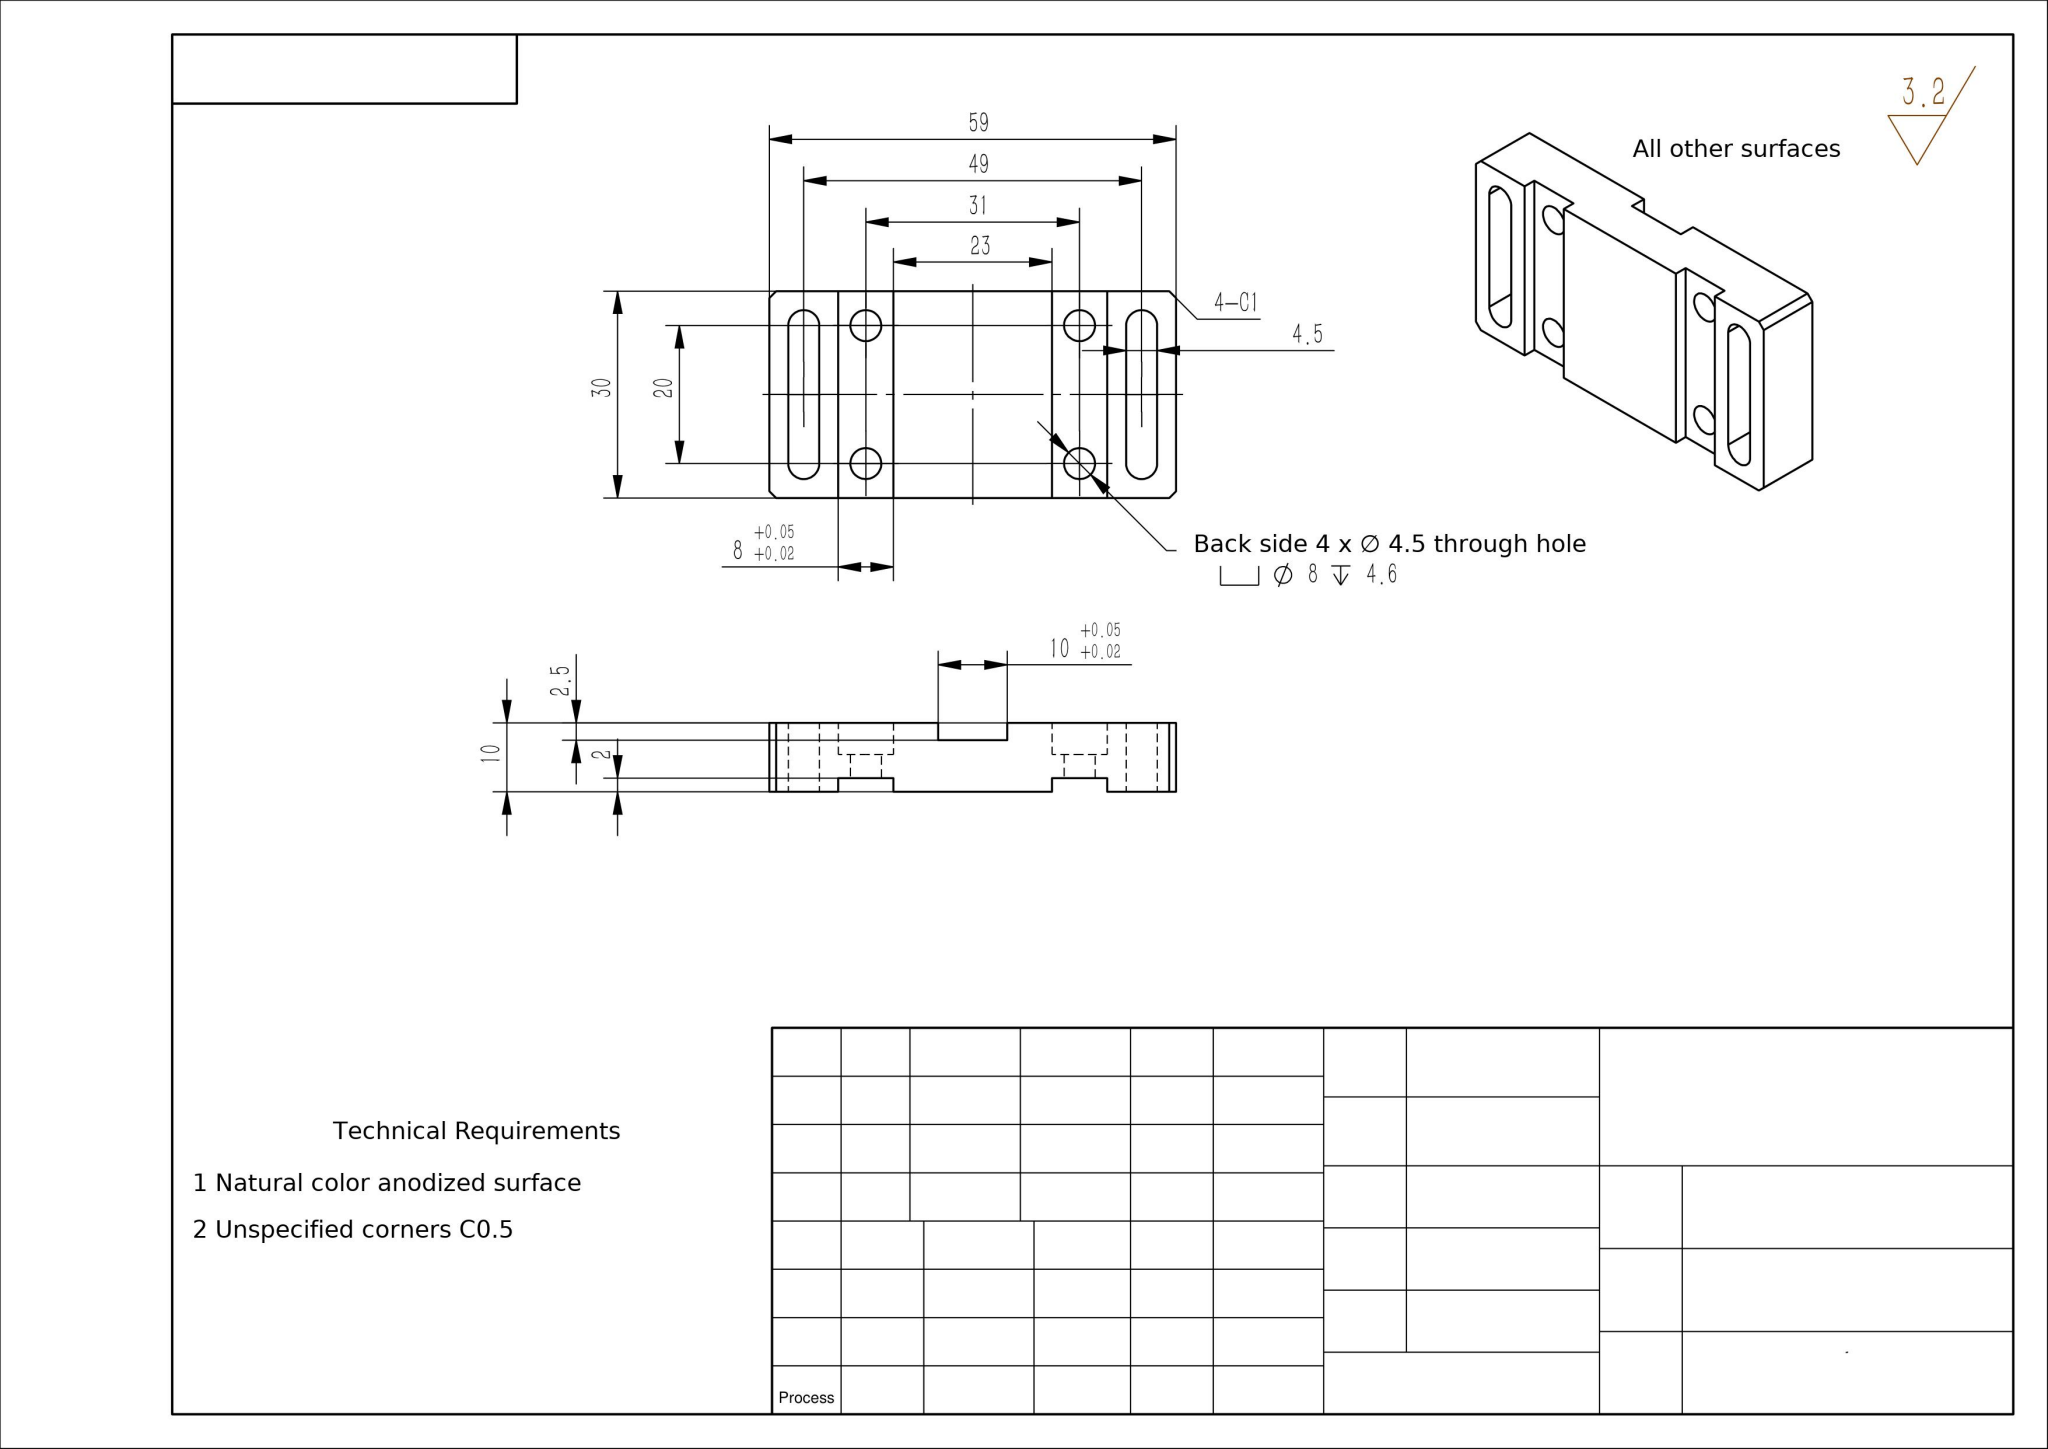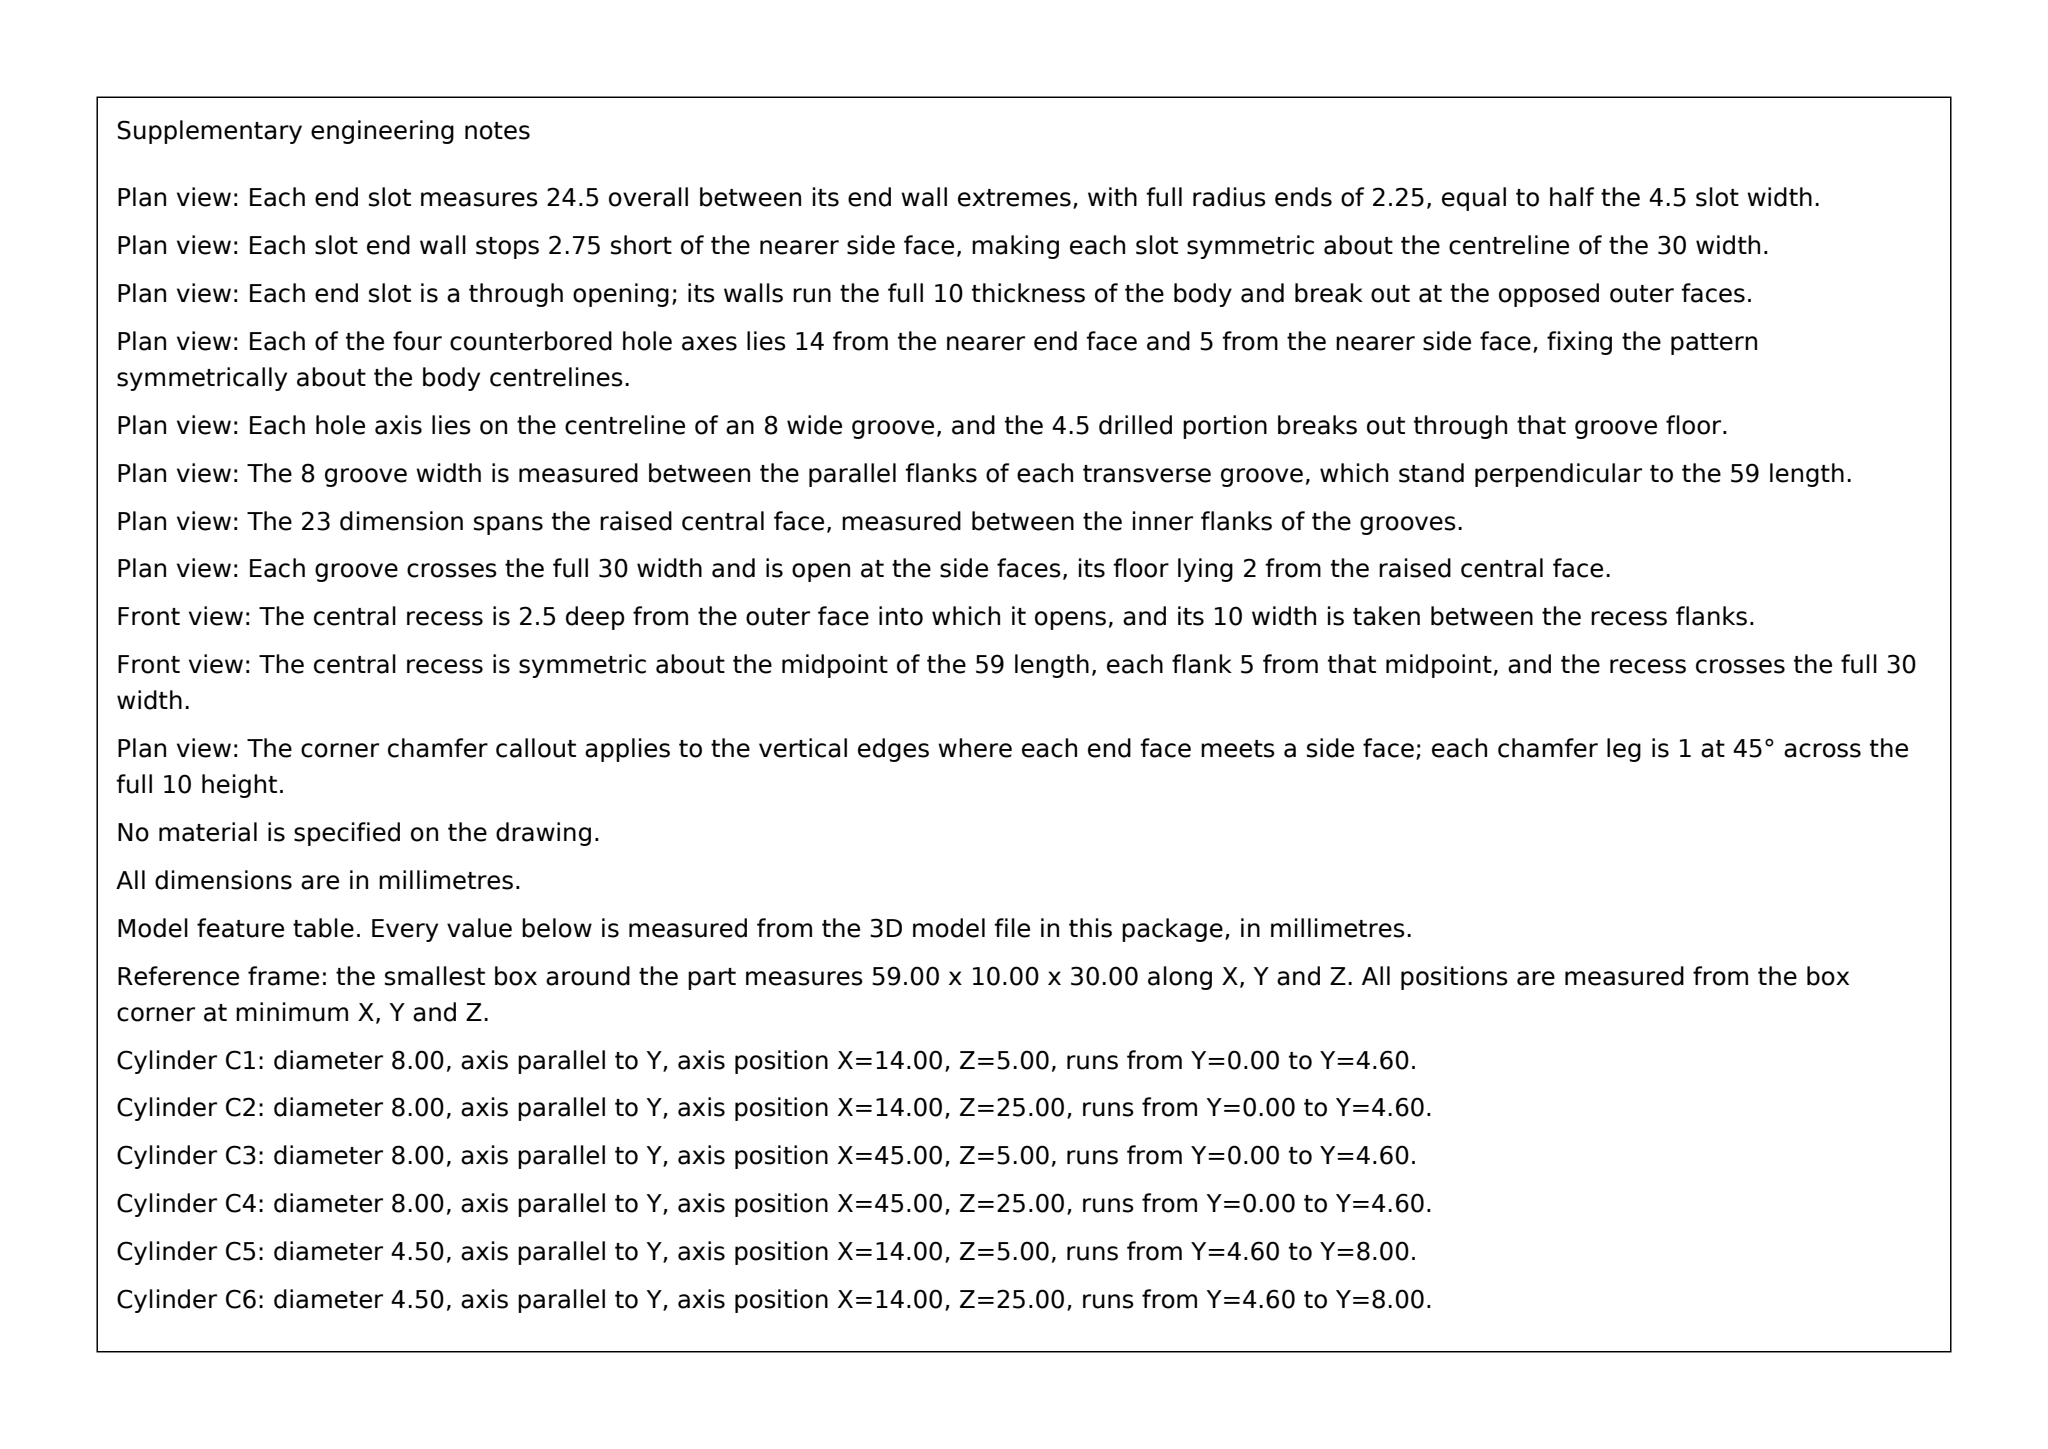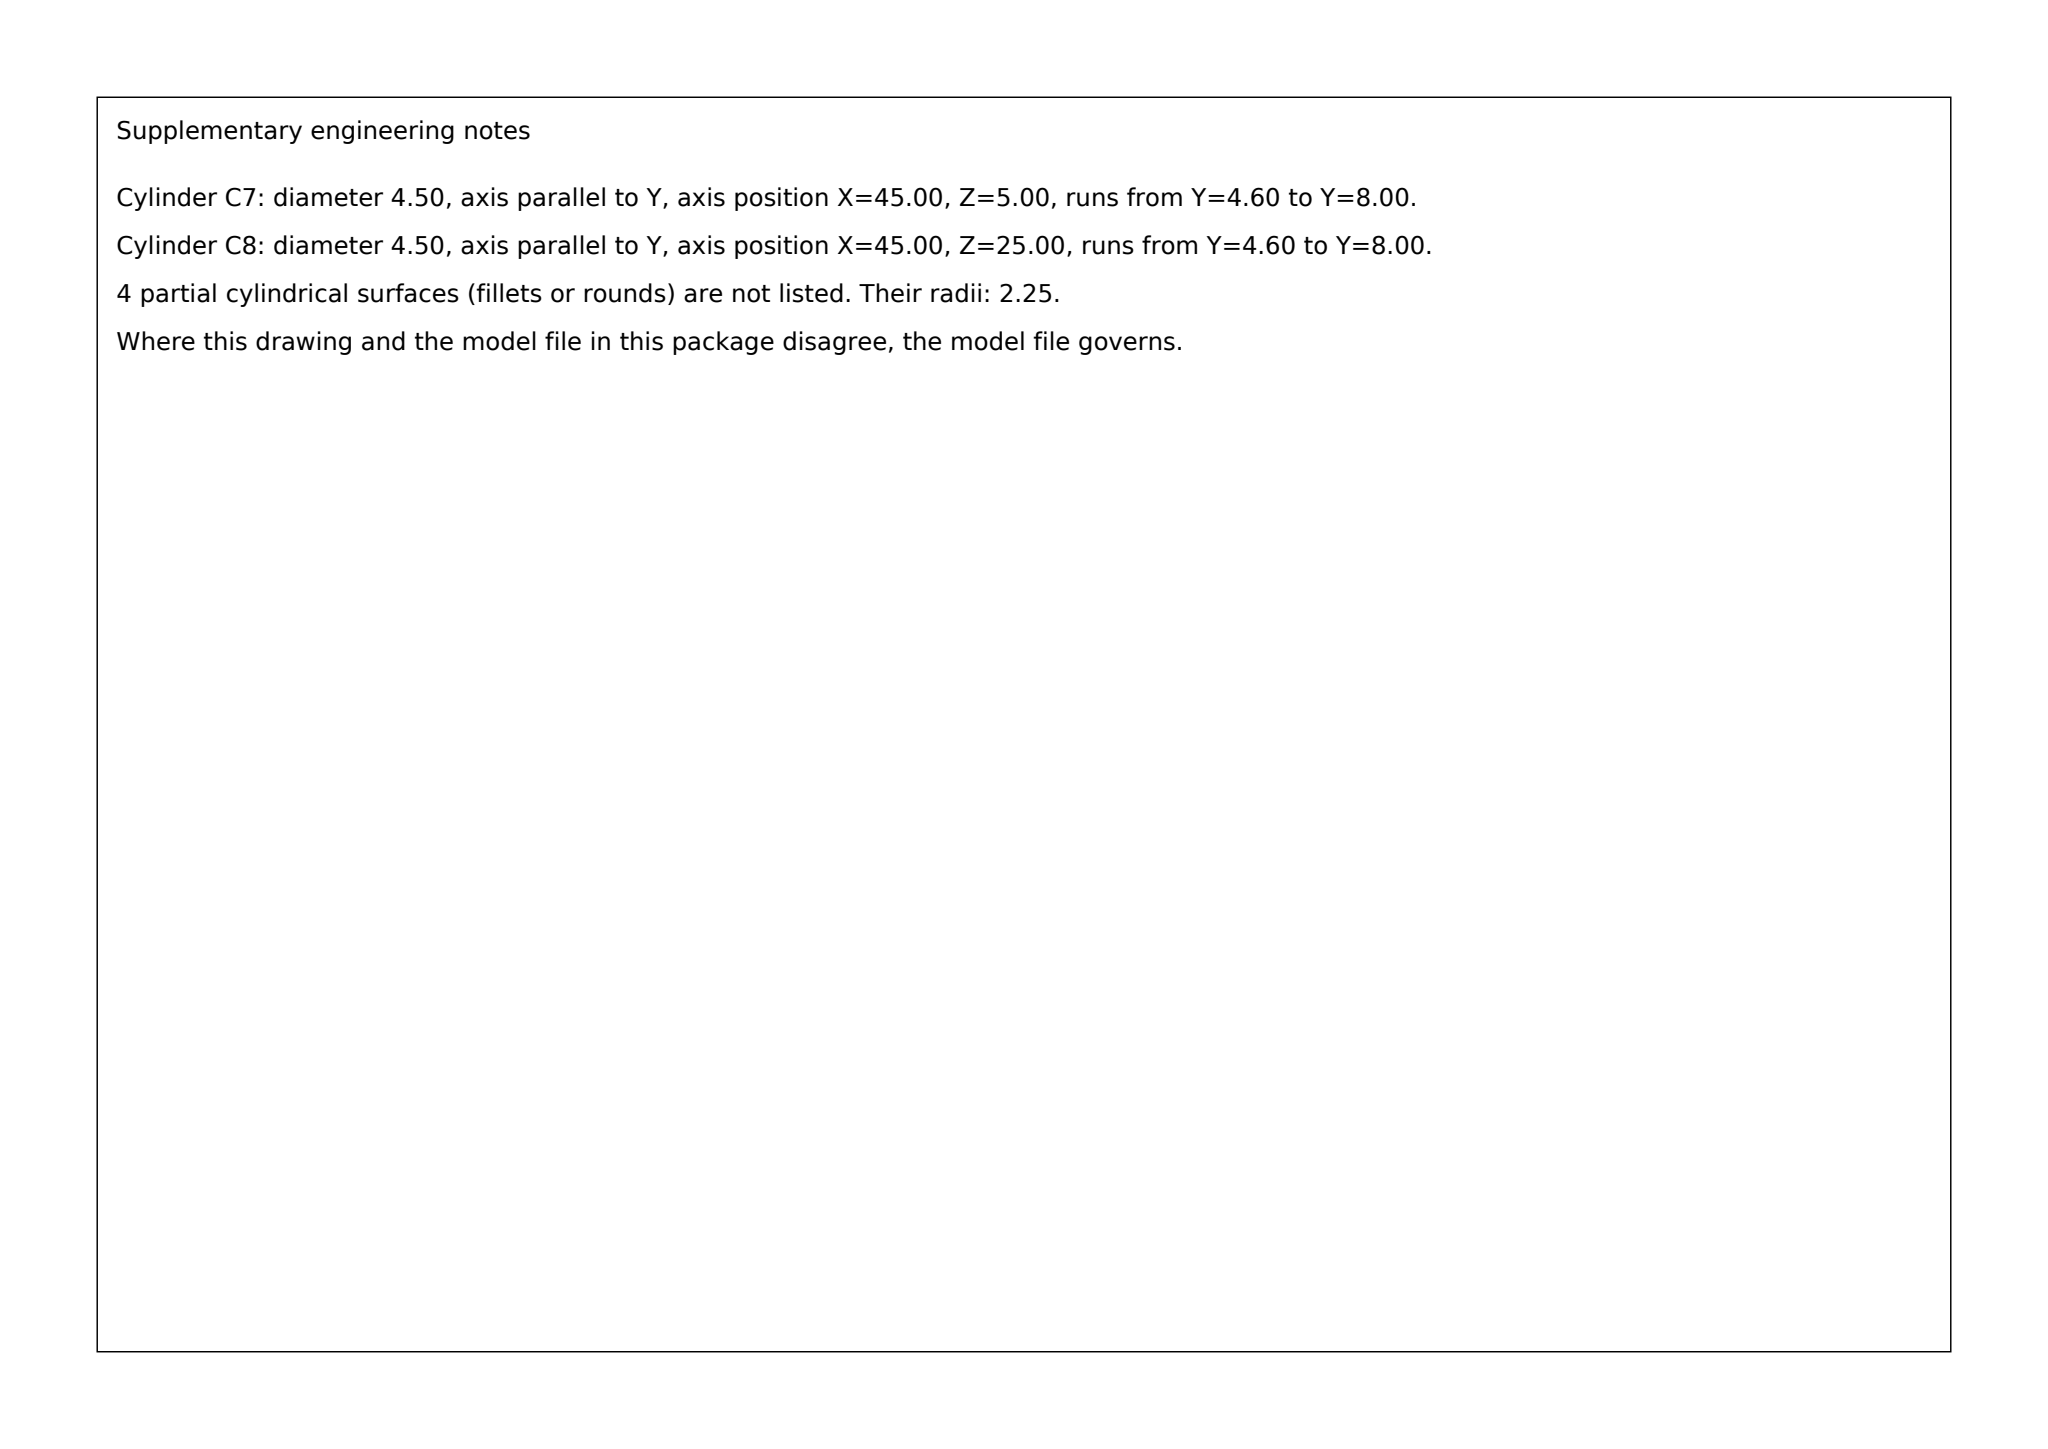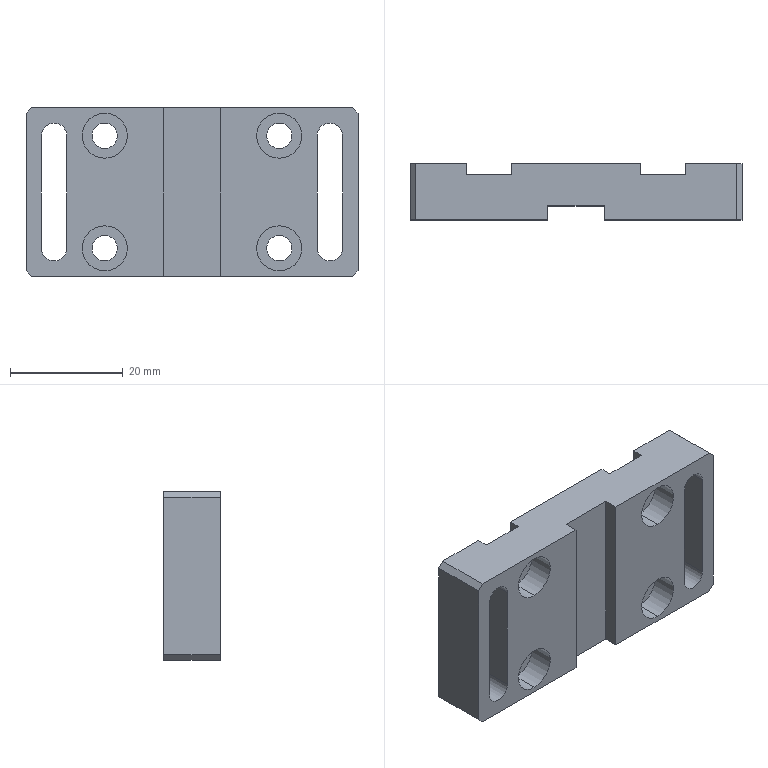Part | SolidWorks | mm | 1 solid | 52 faces | box 59 x 10 x 30 mm | volume 12711 mm3 | plane 30 | cylinder 22 | commonest cylinder face diameters 4.5 x14 8 x8
Drawing notes:
STEP 10 WIDE x 2.5 DP, 24.5 FROM LEFT END FACE | from the solid: Plane y=2.5 spans x 24.5-34.5 (10 wide), 2.5 below y=10 top face; left end face at x=0
build123d program:
from build123d import *

# Parameters (mm, degrees)
SKETCH1_W                                         = 59
SKETCH1_H                                         = 30
BOSS_EXTRUDE1_DEPTH                               = 10
SKETCH2_W                                         = 8
SKETCH2_H                                         = 35.031
CUT_EXTRUDE1_DEPTH                                = 2
CUT_EXTRUDE2_DEPTH                                = 35.572
CHAMFER1_SIZE                                     = 1
HOLE_SIZE_ACCORDING_TO_TYPE_1_OF_HEXA_D           = 4.5
HOLE_SIZE_ACCORDING_TO_TYPE_1_OF_HEXA_CBORE_D     = 8
HOLE_SIZE_ACCORDING_TO_TYPE_1_OF_HEXA_CBORE_DEPTH = 4.6
SKETCH6_W                                         = 10
SKETCH6_H                                         = 5
CUT_EXTRUDE3_DEPTH                                = 44.246


with BuildPart() as part:
    # Sketch1 → Boss-Extrude1 (new body)
    with BuildSketch(Plane(origin=(0, 0, 0), x_dir=(1, 0, 0), z_dir=(0, 1, 0))):
        Rectangle(SKETCH1_W, SKETCH1_H)
    extrude(amount=BOSS_EXTRUDE1_DEPTH)

    # Sketch2 → Cut-Extrude1 (cut)
    with BuildSketch(Plane(origin=(0, 10, 0), x_dir=(1, 0, 0), z_dir=(0, 1, 0))):
        with Locations((15.5, 0.6493)):
            Rectangle(SKETCH2_W, SKETCH2_H)
        with Locations((-15.5, 0.6493)):
            Rectangle(SKETCH2_W, SKETCH2_H)
    extrude(amount=-CUT_EXTRUDE1_DEPTH, mode=Mode.SUBTRACT)

    # Sketch3 → Cut-Extrude2 (cut, through all)
    with BuildSketch(Plane(origin=(0, 10, 0), x_dir=(1, 0, 0), z_dir=(0, 1, 0))):
        with BuildLine():
            Line((-22.25, 10), (-22.25, -10))
            ThreePointArc((-22.25, -10), (-24.5, -12.25), (-26.75, -10))
            Line((-26.75, -10), (-26.75, 10))
            ThreePointArc((-26.75, 10), (-24.5, 12.25), (-22.25, 10))
        make_face()
        with BuildLine():
            Line((22.25, 10), (22.25, -10))
            ThreePointArc((22.25, -10), (24.5, -12.25), (26.75, -10))
            Line((26.75, -10), (26.75, 10))
            ThreePointArc((26.75, 10), (24.5, 12.25), (22.25, 10))
        make_face()
    extrude(amount=-CUT_EXTRUDE2_DEPTH, mode=Mode.SUBTRACT)

    # Chamfer1
    chamfer1_edges = [part.edges().sort_by_distance(p)[0] for p in [
        (29.5, 5, 15),
        (-29.5, 5, 15),
        (-29.5, 5, -15),
        (29.5, 5, -15),
    ]]
    chamfer(chamfer1_edges, length=CHAMFER1_SIZE)

    # Hole Size _ according to_ Type 1 of Hexa (through all)
    with Locations(Plane(origin=(0, 0, 0), x_dir=(-1, 0, 0), z_dir=(0, -1, 0))):
        with Locations((15.5, -10), (15.5, 10), (-15.5, -10), (-15.5, 10)):
            CounterBoreHole(HOLE_SIZE_ACCORDING_TO_TYPE_1_OF_HEXA_D / 2, HOLE_SIZE_ACCORDING_TO_TYPE_1_OF_HEXA_CBORE_D / 2, HOLE_SIZE_ACCORDING_TO_TYPE_1_OF_HEXA_CBORE_DEPTH)

    # Sketch6 → Cut-Extrude3 (cut, through all)
    with BuildSketch(Plane(origin=(0, 0, -15), x_dir=(-1, 0, 0), z_dir=(0, 0, -1))):
        Rectangle(SKETCH6_W, SKETCH6_H)
    extrude(amount=-CUT_EXTRUDE3_DEPTH, mode=Mode.SUBTRACT)


solid = part.part